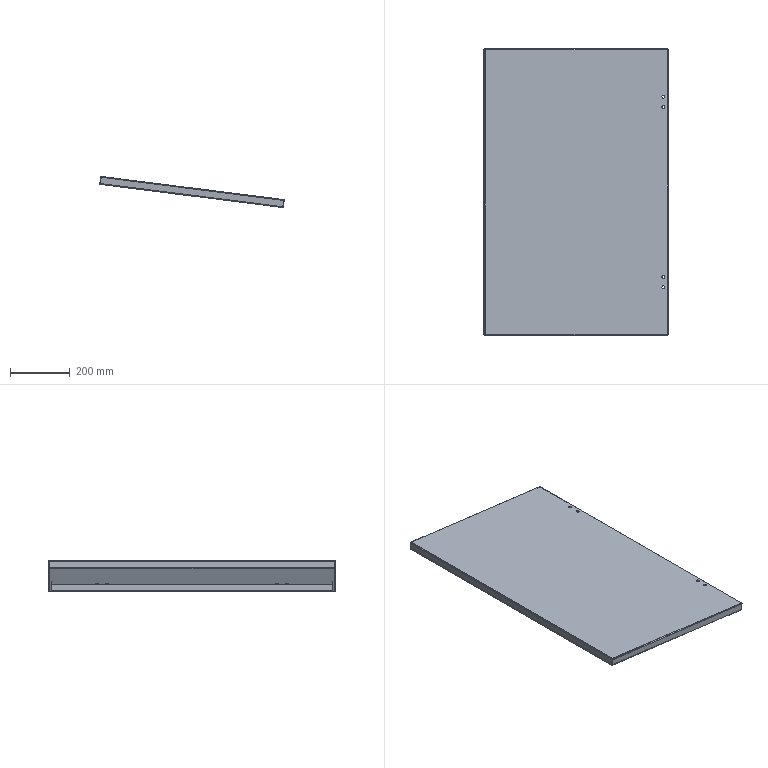Component | SolidWorks | 35RightFrontDoor-1 | 1 solid | 78 faces | volume 1389234 mm3 | plane 38 | cylinder 24 | spline 16 | commonest cylinder face diameters 10 x8 2 x8 6 x8